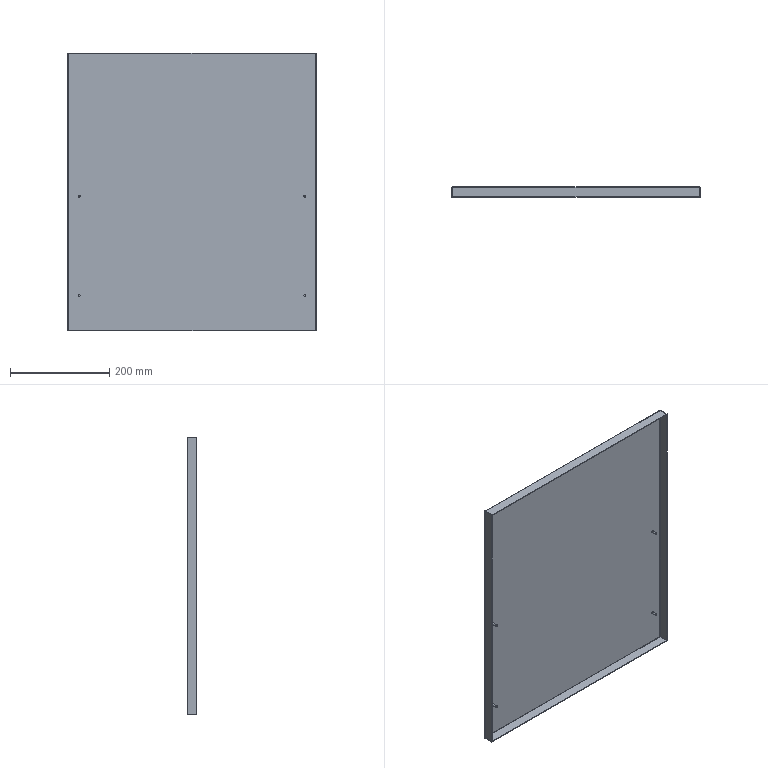Component | SolidWorks | TopPlateWelding-1_TopPlate-1 | 1 solid | 54 faces | volume 477998 mm3 | plane 38 | cylinder 16 | commonest cylinder face diameters 4 x8 3.2 x4 0.2 x4